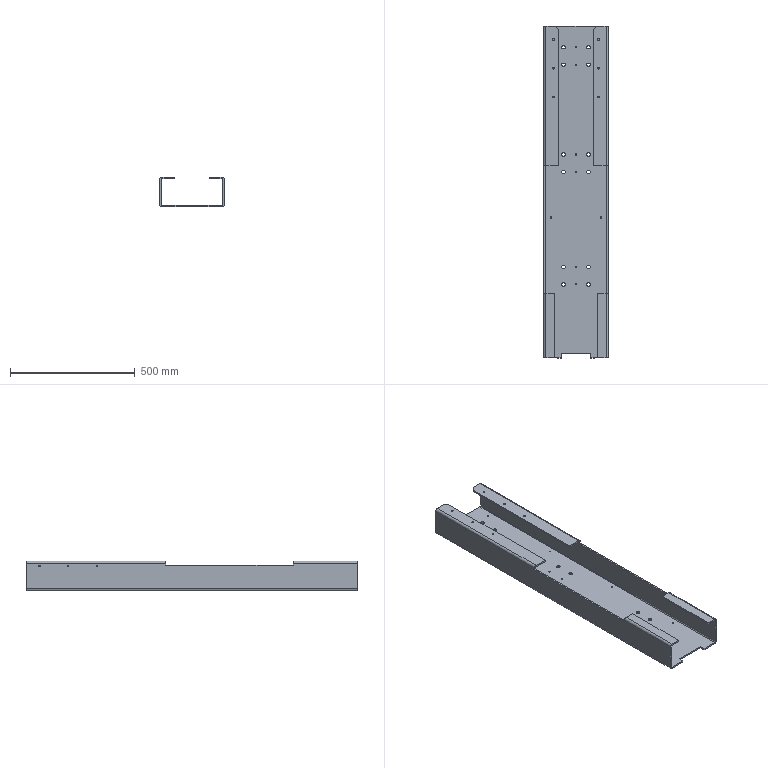Component | SolidWorks | THK-A1001VerticalBeamC-ChannelSteel-1 | 1 solid | 150 faces | volume 4183866 mm3 | cylinder 94 | plane 56 | commonest cylinder face diameters 5 x30 14 x24 4.2 x16 6.8 x12 18 x6 6 x6 | material Q235A